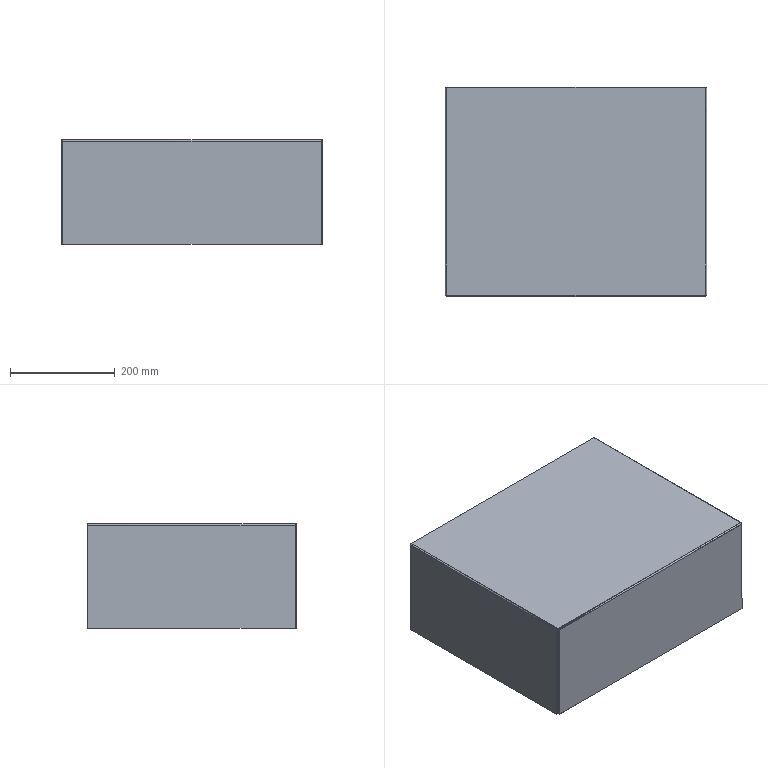Component | SolidWorks | Guard-1 | 1 solid | 30 faces | box 500 x 400 x 200 mm | volume 908561 mm3 | plane 20 | cylinder 6 | spline 4 | commonest cylinder face diameters 5.473 x3 1.473 x3
STEP:
#1=COLOUR_RGB('',0.7922,0.8196,0.9333);
#2=FILL_AREA_STYLE_COLOUR('',#1);
#3=FILL_AREA_STYLE('',(#2));
#4=SURFACE_STYLE_FILL_AREA(#3);
#5=SURFACE_SIDE_STYLE('',(#4));
#6=SURFACE_STYLE_USAGE(.BOTH.,#5);
#7=PRESENTATION_STYLE_ASSIGNMENT((#6));
#8=CARTESIAN_POINT('',(10.744,-9.76,24.528));
#9=VERTEX_POINT('',#8);
#10=CARTESIAN_POINT('',(-8.726,-9.76,24.528));
#11=VERTEX_POINT('',#10);
#12=CARTESIAN_POINT('',(-8.833,-9.76,24.528));
#13=DIRECTION('',(-1.,0.,0.));
#14=VECTOR('',#13,39.37);
#15=LINE('',#12,#14);
#16=EDGE_CURVE('',#9,#11,#15,.T.);
#17=ORIENTED_EDGE('',*,*,#16,.F.);
#18=CARTESIAN_POINT('',(10.744,-25.4,24.528));
#19=VERTEX_POINT('',#18);
#20=CARTESIAN_POINT('',(10.744,-25.401,24.528));
#21=DIRECTION('',(0.,1.,0.));
#22=VECTOR('',#21,39.37);
#23=LINE('',#20,#22);
#24=EDGE_CURVE('',#19,#9,#23,.T.);
#25=ORIENTED_EDGE('',*,*,#24,.F.);
#26=CARTESIAN_POINT('',(-8.726,-25.4,24.528));
#27=VERTEX_POINT('',#26);
#28=CARTESIAN_POINT('',(-8.727,-25.4,24.528));
#29=DIRECTION('',(1.,0.,0.));
#30=VECTOR('',#29,39.37);
#31=LINE('',#28,#30);
#32=EDGE_CURVE('',#27,#19,#31,.T.);
#33=ORIENTED_EDGE('',*,*,#32,.F.);
#34=CARTESIAN_POINT('',(-8.726,-9.76,24.528));
#35=DIRECTION('',(0.,-1.,0.));
#36=VECTOR('',#35,39.37);
#37=LINE('',#34,#36);
#38=EDGE_CURVE('',#11,#27,#37,.T.);
#39=ORIENTED_EDGE('',*,*,#38,.F.);
#40=EDGE_LOOP('',(#17,#25,#33,#39));
#41=FACE_OUTER_BOUND('',#40,.T.);
#42=CARTESIAN_POINT('',(1.009,-17.634,24.528));
#43=DIRECTION('',(0.,0.,-1.));
#44=DIRECTION('',(-1.,0.,0.));
#45=AXIS2_PLACEMENT_3D('',#42,#43,#44);
#46=PLANE('',#45);
#47=ADVANCED_FACE('',(#41),#46,.T.);
#48=CARTESIAN_POINT('',(10.744,-25.4,24.606));
#49=VERTEX_POINT('',#48);
#50=CARTESIAN_POINT('',(10.744,-9.76,24.606));
#51=VERTEX_POINT('',#50);
#52=CARTESIAN_POINT('',(10.744,-25.401,24.606));
#53=DIRECTION('',(0.,1.,0.));
#54=VECTOR('',#53,39.37);
#55=LINE('',#52,#54);
#56=EDGE_CURVE('',#49,#51,#55,.T.);
#57=ORIENTED_EDGE('',*,*,#56,.T.);
#58=CARTESIAN_POINT('',(-8.726,-9.76,24.606));
#59=VERTEX_POINT('',#58);
#60=CARTESIAN_POINT('',(-8.833,-9.76,24.606));
#61=DIRECTION('',(-1.,0.,0.));
#62=VECTOR('',#61,39.37);
#63=LINE('',#60,#62);
#64=EDGE_CURVE('',#51,#59,#63,.T.);
#65=ORIENTED_EDGE('',*,*,#64,.T.);
#66=CARTESIAN_POINT('',(-8.726,-25.4,24.606));
#67=VERTEX_POINT('',#66);
#68=CARTESIAN_POINT('',(-8.726,-9.76,24.606));
#69=DIRECTION('',(0.,-1.,0.));
#70=VECTOR('',#69,39.37);
#71=LINE('',#68,#70);
#72=EDGE_CURVE('',#59,#67,#71,.T.);
#73=ORIENTED_EDGE('',*,*,#72,.T.);
#74=CARTESIAN_POINT('',(-8.727,-25.4,24.606));
#75=DIRECTION('',(1.,0.,0.));
#76=VECTOR('',#75,39.37);
#77=LINE('',#74,#76);
#78=EDGE_CURVE('',#67,#49,#77,.T.);
#79=ORIENTED_EDGE('',*,*,#78,.T.);
#80=EDGE_LOOP('',(#57,#65,#73,#79));
#81=FACE_OUTER_BOUND('',#80,.T.);
#82=CARTESIAN_POINT('',(1.009,-17.634,24.606));
#83=DIRECTION('',(0.,0.,-1.));
#84=DIRECTION('',(-1.,0.,0.));
#85=AXIS2_PLACEMENT_3D('',#82,#83,#84);
#86=PLANE('',#85);
#87=ADVANCED_FACE('',(#81),#86,.F.);
#88=CARTESIAN_POINT('',(10.744,-9.76,24.528));
#89=DIRECTION('',(0.,0.,1.));
#90=VECTOR('',#89,39.37);
#91=LINE('',#88,#90);
#92=EDGE_CURVE('',#9,#51,#91,.T.);
#93=ORIENTED_EDGE('',*,*,#92,.F.);
#94=ORIENTED_EDGE('',*,*,#16,.T.);
#95=CARTESIAN_POINT('',(-8.726,-9.76,24.528));
#96=DIRECTION('',(0.,0.,1.));
#97=VECTOR('',#96,39.37);
#98=LINE('',#95,#97);
#99=EDGE_CURVE('',#11,#59,#98,.T.);
#100=ORIENTED_EDGE('',*,*,#99,.T.);
#101=ORIENTED_EDGE('',*,*,#64,.F.);
#102=EDGE_LOOP('',(#93,#94,#100,#101));
#103=FACE_OUTER_BOUND('',#102,.T.);
#104=CARTESIAN_POINT('',(-8.833,-9.76,24.528));
#105=DIRECTION('',(0.,1.,0.));
#106=DIRECTION('',(0.,0.,1.));
#107=AXIS2_PLACEMENT_3D('',#104,#105,#106);
#108=PLANE('',#107);
#109=ADVANCED_FACE('',(#103),#108,.T.);
#110=CARTESIAN_POINT('',(-8.833,-25.401,24.499));
#111=VERTEX_POINT('',#110);
#112=CARTESIAN_POINT('',(-8.755,-25.401,24.499));
#113=VERTEX_POINT('',#112);
#114=CARTESIAN_POINT('',(-8.755,-25.401,24.499));
#115=DIRECTION('',(1.,0.,-0.));
#116=VECTOR('',#115,39.37);
#117=LINE('',#114,#116);
#118=EDGE_CURVE('',#111,#113,#117,.T.);
#119=ORIENTED_EDGE('',*,*,#118,.T.);
#120=CARTESIAN_POINT('',(-8.726,-25.4,24.528));
#121=CARTESIAN_POINT('',(-8.733,-25.4,24.528));
#122=CARTESIAN_POINT('',(-8.741,-25.401,24.524));
#123=CARTESIAN_POINT('',(-8.752,-25.401,24.514));
#124=CARTESIAN_POINT('',(-8.755,-25.401,24.506));
#125=CARTESIAN_POINT('',(-8.755,-25.401,24.499));
#126=B_SPLINE_CURVE_WITH_KNOTS('',3,(#120,#121,#122,#123,#124,#125),.UNSPECIFIED.,.F.,.F.,(4,2,4),(0.,0.5,1.),.UNSPECIFIED.);
#127=EDGE_CURVE('',#27,#113,#126,.T.);
#128=ORIENTED_EDGE('',*,*,#127,.F.);
#129=CARTESIAN_POINT('',(-8.726,-25.4,24.528));
#130=DIRECTION('',(0.,0.,1.));
#131=VECTOR('',#130,39.37);
#132=LINE('',#129,#131);
#133=EDGE_CURVE('',#27,#67,#132,.T.);
#134=ORIENTED_EDGE('',*,*,#133,.T.);
#135=CARTESIAN_POINT('',(-8.726,-25.4,24.606));
#136=CARTESIAN_POINT('',(-8.74,-25.4,24.606));
#137=CARTESIAN_POINT('',(-8.754,-25.4,24.603));
#138=CARTESIAN_POINT('',(-8.78,-25.401,24.593));
#139=CARTESIAN_POINT('',(-8.792,-25.401,24.585));
#140=CARTESIAN_POINT('',(-8.812,-25.401,24.565));
#141=CARTESIAN_POINT('',(-8.82,-25.401,24.553));
#142=CARTESIAN_POINT('',(-8.831,-25.401,24.527));
#143=CARTESIAN_POINT('',(-8.833,-25.401,24.513));
#144=CARTESIAN_POINT('',(-8.833,-25.401,24.499));
#145=B_SPLINE_CURVE_WITH_KNOTS('',3,(#135,#136,#137,#138,#139,#140,#141,#142,#143,#144),.UNSPECIFIED.,.F.,.F.,(4,2,2,2,4),(0.,0.25,0.5,0.75,1.),.UNSPECIFIED.);
#146=EDGE_CURVE('',#67,#111,#145,.T.);
#147=ORIENTED_EDGE('',*,*,#146,.T.);
#148=EDGE_LOOP('',(#119,#128,#134,#147));
#149=FACE_OUTER_BOUND('',#148,.T.);
#150=CARTESIAN_POINT('',(-8.726,-25.4,24.607));
#151=CARTESIAN_POINT('',(-8.74,-25.4,24.607));
#152=CARTESIAN_POINT('',(-8.754,-25.4,24.604));
#153=CARTESIAN_POINT('',(-8.78,-25.401,24.593));
#154=CARTESIAN_POINT('',(-8.792,-25.401,24.585));
#155=CARTESIAN_POINT('',(-8.813,-25.401,24.565));
#156=CARTESIAN_POINT('',(-8.821,-25.401,24.553));
#157=CARTESIAN_POINT('',(-8.831,-25.401,24.527));
#158=CARTESIAN_POINT('',(-8.834,-25.401,24.513));
#159=CARTESIAN_POINT('',(-8.834,-25.401,24.499));
#160=CARTESIAN_POINT('',(-8.726,-25.4,24.606));
#161=CARTESIAN_POINT('',(-8.74,-25.4,24.606));
#162=CARTESIAN_POINT('',(-8.754,-25.4,24.603));
#163=CARTESIAN_POINT('',(-8.78,-25.401,24.593));
#164=CARTESIAN_POINT('',(-8.792,-25.401,24.585));
#165=CARTESIAN_POINT('',(-8.812,-25.401,24.565));
#166=CARTESIAN_POINT('',(-8.82,-25.401,24.553));
#167=CARTESIAN_POINT('',(-8.831,-25.401,24.527));
#168=CARTESIAN_POINT('',(-8.833,-25.401,24.513));
#169=CARTESIAN_POINT('',(-8.833,-25.401,24.499));
#170=CARTESIAN_POINT('',(-8.726,-25.4,24.528));
#171=CARTESIAN_POINT('',(-8.73,-25.4,24.528));
#172=CARTESIAN_POINT('',(-8.733,-25.4,24.527));
#173=CARTESIAN_POINT('',(-8.74,-25.401,24.524));
#174=CARTESIAN_POINT('',(-8.744,-25.401,24.522));
#175=CARTESIAN_POINT('',(-8.749,-25.401,24.516));
#176=CARTESIAN_POINT('',(-8.751,-25.401,24.513));
#177=CARTESIAN_POINT('',(-8.754,-25.401,24.506));
#178=CARTESIAN_POINT('',(-8.755,-25.401,24.502));
#179=CARTESIAN_POINT('',(-8.755,-25.401,24.499));
#180=CARTESIAN_POINT('',(-8.726,-25.4,24.527));
#181=CARTESIAN_POINT('',(-8.729,-25.4,24.527));
#182=CARTESIAN_POINT('',(-8.733,-25.4,24.526));
#183=CARTESIAN_POINT('',(-8.74,-25.401,24.523));
#184=CARTESIAN_POINT('',(-8.743,-25.401,24.521));
#185=CARTESIAN_POINT('',(-8.748,-25.401,24.516));
#186=CARTESIAN_POINT('',(-8.75,-25.401,24.513));
#187=CARTESIAN_POINT('',(-8.753,-25.401,24.506));
#188=CARTESIAN_POINT('',(-8.754,-25.401,24.502));
#189=CARTESIAN_POINT('',(-8.754,-25.401,24.499));
#190=B_SPLINE_SURFACE_WITH_KNOTS('',1,3,((#150,#151,#152,#153,#154,#155,#156,#157,#158,#159),(#160,#161,#162,#163,#164,#165,#166,#167,#168,#169),(#170,#171,#172,#173,#174,#175,#176,#177,#178,#179),(#180,#181,#182,#183,#184,#185,#186,#187,#188,#189)),.UNSPECIFIED.,.F.,.F.,.F.,(2,1,1,2),(4,2,2,2,4),(-0.01,0.,1.,1.01),(0.,0.25,0.5,0.75,1.),.UNSPECIFIED.);
#191=ADVANCED_FACE('',(#149),#190,.F.);
#192=CARTESIAN_POINT('',(-8.755,-9.76,24.499));
#193=VERTEX_POINT('',#192);
#194=CARTESIAN_POINT('',(-8.726,-9.76,24.499));
#195=DIRECTION('',(0.,1.,0.));
#196=DIRECTION('',(0.,0.,1.));
#197=AXIS2_PLACEMENT_3D('',#194,#195,#196);
#198=CIRCLE('',#197,0.029);
#199=EDGE_CURVE('',#193,#11,#198,.T.);
#200=ORIENTED_EDGE('',*,*,#199,.F.);
#201=CARTESIAN_POINT('',(-8.833,-9.76,24.499));
#202=VERTEX_POINT('',#201);
#203=CARTESIAN_POINT('',(-8.755,-9.76,24.499));
#204=DIRECTION('',(-1.,0.,0.));
#205=VECTOR('',#204,39.37);
#206=LINE('',#203,#205);
#207=EDGE_CURVE('',#193,#202,#206,.T.);
#208=ORIENTED_EDGE('',*,*,#207,.T.);
#209=CARTESIAN_POINT('',(-8.726,-9.76,24.499));
#210=DIRECTION('',(0.,1.,0.));
#211=DIRECTION('',(0.,0.,1.));
#212=AXIS2_PLACEMENT_3D('',#209,#210,#211);
#213=CIRCLE('',#212,0.1077);
#214=EDGE_CURVE('',#202,#59,#213,.T.);
#215=ORIENTED_EDGE('',*,*,#214,.T.);
#216=ORIENTED_EDGE('',*,*,#99,.F.);
#217=EDGE_LOOP('',(#200,#208,#215,#216));
#218=FACE_OUTER_BOUND('',#217,.T.);
#219=CARTESIAN_POINT('',(-8.726,-9.76,24.499));
#220=DIRECTION('',(0.,-1.,0.));
#221=DIRECTION('',(0.,0.,-1.));
#222=AXIS2_PLACEMENT_3D('',#219,#220,#221);
#223=PLANE('',#222);
#224=ADVANCED_FACE('',(#218),#223,.F.);
#225=ORIENTED_EDGE('',*,*,#72,.F.);
#226=ORIENTED_EDGE('',*,*,#214,.F.);
#227=CARTESIAN_POINT('',(-8.833,-17.634,24.499));
#228=DIRECTION('',(0.,1.,0.));
#229=VECTOR('',#228,39.37);
#230=LINE('',#227,#229);
#231=EDGE_CURVE('',#111,#202,#230,.T.);
#232=ORIENTED_EDGE('',*,*,#231,.F.);
#233=ORIENTED_EDGE('',*,*,#146,.F.);
#234=EDGE_LOOP('',(#225,#226,#232,#233));
#235=FACE_OUTER_BOUND('',#234,.T.);
#236=CARTESIAN_POINT('',(-8.726,-9.76,24.499));
#237=DIRECTION('',(0.,1.,0.));
#238=DIRECTION('',(-1.,0.,0.));
#239=AXIS2_PLACEMENT_3D('',#236,#237,#238);
#240=CYLINDRICAL_SURFACE('',#239,0.1077);
#241=ADVANCED_FACE('',(#235),#240,.T.);
#242=ORIENTED_EDGE('',*,*,#38,.T.);
#243=ORIENTED_EDGE('',*,*,#127,.T.);
#244=CARTESIAN_POINT('',(-8.755,-25.508,24.499));
#245=DIRECTION('',(0.,1.,0.));
#246=VECTOR('',#245,39.37);
#247=LINE('',#244,#246);
#248=EDGE_CURVE('',#113,#193,#247,.T.);
#249=ORIENTED_EDGE('',*,*,#248,.T.);
#250=ORIENTED_EDGE('',*,*,#199,.T.);
#251=EDGE_LOOP('',(#242,#243,#249,#250));
#252=FACE_OUTER_BOUND('',#251,.T.);
#253=CARTESIAN_POINT('',(-8.726,-9.76,24.499));
#254=DIRECTION('',(0.,1.,0.));
#255=DIRECTION('',(-1.,0.,0.));
#256=AXIS2_PLACEMENT_3D('',#253,#254,#255);
#257=CYLINDRICAL_SURFACE('',#256,0.029);
#258=ADVANCED_FACE('',(#252),#257,.F.);
#259=CARTESIAN_POINT('',(-8.755,-25.401,16.732));
#260=VERTEX_POINT('',#259);
#261=CARTESIAN_POINT('',(-8.833,-25.401,16.732));
#262=VERTEX_POINT('',#261);
#263=CARTESIAN_POINT('',(-8.833,-25.401,16.732));
#264=DIRECTION('',(-1.,-0.,0.));
#265=VECTOR('',#264,39.37);
#266=LINE('',#263,#265);
#267=EDGE_CURVE('',#260,#262,#266,.T.);
#268=ORIENTED_EDGE('',*,*,#267,.F.);
#269=CARTESIAN_POINT('',(-8.755,-25.401,24.606));
#270=DIRECTION('',(-0.,0.,-1.));
#271=VECTOR('',#270,39.37);
#272=LINE('',#269,#271);
#273=EDGE_CURVE('',#113,#260,#272,.T.);
#274=ORIENTED_EDGE('',*,*,#273,.F.);
#275=ORIENTED_EDGE('',*,*,#118,.F.);
#276=CARTESIAN_POINT('',(-8.833,-25.401,24.606));
#277=DIRECTION('',(0.,-0.,1.));
#278=VECTOR('',#277,39.37);
#279=LINE('',#276,#278);
#280=EDGE_CURVE('',#262,#111,#279,.T.);
#281=ORIENTED_EDGE('',*,*,#280,.F.);
#282=EDGE_LOOP('',(#268,#274,#275,#281));
#283=FACE_OUTER_BOUND('',#282,.T.);
#284=CARTESIAN_POINT('',(-8.755,-25.401,24.528));
#285=DIRECTION('',(-0.,-1.,-0.));
#286=DIRECTION('',(0.,0.,-1.));
#287=AXIS2_PLACEMENT_3D('',#284,#285,#286);
#288=PLANE('',#287);
#289=ADVANCED_FACE('',(#283),#288,.T.);
#290=CARTESIAN_POINT('',(-8.833,-9.76,16.732));
#291=VERTEX_POINT('',#290);
#292=CARTESIAN_POINT('',(-8.833,-9.76,16.732));
#293=DIRECTION('',(0.,1.,0.));
#294=VECTOR('',#293,39.37);
#295=LINE('',#292,#294);
#296=EDGE_CURVE('',#262,#291,#295,.T.);
#297=ORIENTED_EDGE('',*,*,#296,.F.);
#298=ORIENTED_EDGE('',*,*,#280,.T.);
#299=ORIENTED_EDGE('',*,*,#231,.T.);
#300=CARTESIAN_POINT('',(-8.833,-9.76,24.528));
#301=DIRECTION('',(0.,0.,1.));
#302=VECTOR('',#301,39.37);
#303=LINE('',#300,#302);
#304=EDGE_CURVE('',#291,#202,#303,.T.);
#305=ORIENTED_EDGE('',*,*,#304,.F.);
#306=EDGE_LOOP('',(#297,#298,#299,#305));
#307=FACE_OUTER_BOUND('',#306,.T.);
#308=CARTESIAN_POINT('',(-8.833,-17.634,24.606));
#309=DIRECTION('',(-1.,0.,0.));
#310=DIRECTION('',(0.,0.,1.));
#311=AXIS2_PLACEMENT_3D('',#308,#309,#310);
#312=PLANE('',#311);
#313=ADVANCED_FACE('',(#307),#312,.T.);
#314=ORIENTED_EDGE('',*,*,#273,.T.);
#315=CARTESIAN_POINT('',(-8.755,-9.76,16.732));
#316=VERTEX_POINT('',#315);
#317=CARTESIAN_POINT('',(-8.755,-17.634,16.732));
#318=DIRECTION('',(0.,1.,0.));
#319=VECTOR('',#318,39.37);
#320=LINE('',#317,#319);
#321=EDGE_CURVE('',#260,#316,#320,.T.);
#322=ORIENTED_EDGE('',*,*,#321,.T.);
#323=CARTESIAN_POINT('',(-8.755,-9.76,24.606));
#324=DIRECTION('',(0.,0.,1.));
#325=VECTOR('',#324,39.37);
#326=LINE('',#323,#325);
#327=EDGE_CURVE('',#316,#193,#326,.T.);
#328=ORIENTED_EDGE('',*,*,#327,.T.);
#329=ORIENTED_EDGE('',*,*,#248,.F.);
#330=EDGE_LOOP('',(#314,#322,#328,#329));
#331=FACE_OUTER_BOUND('',#330,.T.);
#332=CARTESIAN_POINT('',(-8.755,-17.634,24.606));
#333=DIRECTION('',(-1.,0.,0.));
#334=DIRECTION('',(0.,0.,1.));
#335=AXIS2_PLACEMENT_3D('',#332,#333,#334);
#336=PLANE('',#335);
#337=ADVANCED_FACE('',(#331),#336,.F.);
#338=ORIENTED_EDGE('',*,*,#321,.F.);
#339=ORIENTED_EDGE('',*,*,#267,.T.);
#340=ORIENTED_EDGE('',*,*,#296,.T.);
#341=CARTESIAN_POINT('',(-8.833,-9.76,16.732));
#342=DIRECTION('',(1.,0.,-0.));
#343=VECTOR('',#342,39.37);
#344=LINE('',#341,#343);
#345=EDGE_CURVE('',#291,#316,#344,.T.);
#346=ORIENTED_EDGE('',*,*,#345,.T.);
#347=EDGE_LOOP('',(#338,#339,#340,#346));
#348=FACE_OUTER_BOUND('',#347,.T.);
#349=CARTESIAN_POINT('',(-8.833,-9.76,16.732));
#350=DIRECTION('',(-0.,0.,-1.));
#351=DIRECTION('',(-1.,0.,0.));
#352=AXIS2_PLACEMENT_3D('',#349,#350,#351);
#353=PLANE('',#352);
#354=ADVANCED_FACE('',(#348),#353,.T.);
#355=ORIENTED_EDGE('',*,*,#304,.T.);
#356=ORIENTED_EDGE('',*,*,#207,.F.);
#357=ORIENTED_EDGE('',*,*,#327,.F.);
#358=ORIENTED_EDGE('',*,*,#345,.F.);
#359=EDGE_LOOP('',(#355,#356,#357,#358));
#360=FACE_OUTER_BOUND('',#359,.T.);
#361=CARTESIAN_POINT('',(-8.833,-9.76,24.528));
#362=DIRECTION('',(0.,1.,0.));
#363=DIRECTION('',(0.,0.,1.));
#364=AXIS2_PLACEMENT_3D('',#361,#362,#363);
#365=PLANE('',#364);
#366=ADVANCED_FACE('',(#360),#365,.T.);
#367=CARTESIAN_POINT('',(10.745,-25.508,24.499));
#368=VERTEX_POINT('',#367);
#369=CARTESIAN_POINT('',(10.745,-25.429,24.499));
#370=VERTEX_POINT('',#369);
#371=CARTESIAN_POINT('',(10.745,-25.429,24.499));
#372=DIRECTION('',(0.,1.,-0.));
#373=VECTOR('',#372,39.37);
#374=LINE('',#371,#373);
#375=EDGE_CURVE('',#368,#370,#374,.T.);
#376=ORIENTED_EDGE('',*,*,#375,.T.);
#377=CARTESIAN_POINT('',(10.744,-25.4,24.528));
#378=CARTESIAN_POINT('',(10.744,-25.408,24.528));
#379=CARTESIAN_POINT('',(10.744,-25.415,24.524));
#380=CARTESIAN_POINT('',(10.745,-25.426,24.514));
#381=CARTESIAN_POINT('',(10.745,-25.429,24.506));
#382=CARTESIAN_POINT('',(10.745,-25.429,24.499));
#383=B_SPLINE_CURVE_WITH_KNOTS('',3,(#377,#378,#379,#380,#381,#382),.UNSPECIFIED.,.F.,.F.,(4,2,4),(0.,0.5,1.),.UNSPECIFIED.);
#384=EDGE_CURVE('',#19,#370,#383,.T.);
#385=ORIENTED_EDGE('',*,*,#384,.F.);
#386=CARTESIAN_POINT('',(10.744,-25.4,24.528));
#387=DIRECTION('',(0.,0.,1.));
#388=VECTOR('',#387,39.37);
#389=LINE('',#386,#388);
#390=EDGE_CURVE('',#19,#49,#389,.T.);
#391=ORIENTED_EDGE('',*,*,#390,.T.);
#392=CARTESIAN_POINT('',(10.744,-25.4,24.606));
#393=CARTESIAN_POINT('',(10.744,-25.414,24.606));
#394=CARTESIAN_POINT('',(10.744,-25.428,24.603));
#395=CARTESIAN_POINT('',(10.744,-25.454,24.593));
#396=CARTESIAN_POINT('',(10.744,-25.466,24.585));
#397=CARTESIAN_POINT('',(10.744,-25.486,24.565));
#398=CARTESIAN_POINT('',(10.745,-25.494,24.553));
#399=CARTESIAN_POINT('',(10.745,-25.505,24.527));
#400=CARTESIAN_POINT('',(10.745,-25.508,24.513));
#401=CARTESIAN_POINT('',(10.745,-25.508,24.499));
#402=B_SPLINE_CURVE_WITH_KNOTS('',3,(#392,#393,#394,#395,#396,#397,#398,#399,#400,#401),.UNSPECIFIED.,.F.,.F.,(4,2,2,2,4),(0.,0.25,0.5,0.75,1.),.UNSPECIFIED.);
#403=EDGE_CURVE('',#49,#368,#402,.T.);
#404=ORIENTED_EDGE('',*,*,#403,.T.);
#405=EDGE_LOOP('',(#376,#385,#391,#404));
#406=FACE_OUTER_BOUND('',#405,.T.);
#407=CARTESIAN_POINT('',(10.744,-25.4,24.607));
#408=CARTESIAN_POINT('',(10.744,-25.414,24.607));
#409=CARTESIAN_POINT('',(10.744,-25.429,24.604));
#410=CARTESIAN_POINT('',(10.744,-25.455,24.593));
#411=CARTESIAN_POINT('',(10.744,-25.467,24.585));
#412=CARTESIAN_POINT('',(10.744,-25.487,24.565));
#413=CARTESIAN_POINT('',(10.745,-25.495,24.553));
#414=CARTESIAN_POINT('',(10.745,-25.506,24.527));
#415=CARTESIAN_POINT('',(10.745,-25.509,24.513));
#416=CARTESIAN_POINT('',(10.745,-25.509,24.499));
#417=CARTESIAN_POINT('',(10.744,-25.4,24.606));
#418=CARTESIAN_POINT('',(10.744,-25.414,24.606));
#419=CARTESIAN_POINT('',(10.744,-25.428,24.603));
#420=CARTESIAN_POINT('',(10.744,-25.454,24.593));
#421=CARTESIAN_POINT('',(10.744,-25.466,24.585));
#422=CARTESIAN_POINT('',(10.744,-25.486,24.565));
#423=CARTESIAN_POINT('',(10.745,-25.494,24.553));
#424=CARTESIAN_POINT('',(10.745,-25.505,24.527));
#425=CARTESIAN_POINT('',(10.745,-25.508,24.513));
#426=CARTESIAN_POINT('',(10.745,-25.508,24.499));
#427=CARTESIAN_POINT('',(10.744,-25.4,24.528));
#428=CARTESIAN_POINT('',(10.744,-25.404,24.528));
#429=CARTESIAN_POINT('',(10.744,-25.408,24.527));
#430=CARTESIAN_POINT('',(10.744,-25.415,24.524));
#431=CARTESIAN_POINT('',(10.744,-25.418,24.522));
#432=CARTESIAN_POINT('',(10.744,-25.423,24.516));
#433=CARTESIAN_POINT('',(10.745,-25.425,24.513));
#434=CARTESIAN_POINT('',(10.745,-25.428,24.506));
#435=CARTESIAN_POINT('',(10.745,-25.429,24.502));
#436=CARTESIAN_POINT('',(10.745,-25.429,24.499));
#437=CARTESIAN_POINT('',(10.744,-25.4,24.527));
#438=CARTESIAN_POINT('',(10.744,-25.404,24.527));
#439=CARTESIAN_POINT('',(10.744,-25.408,24.526));
#440=CARTESIAN_POINT('',(10.744,-25.414,24.523));
#441=CARTESIAN_POINT('',(10.744,-25.417,24.521));
#442=CARTESIAN_POINT('',(10.744,-25.423,24.516));
#443=CARTESIAN_POINT('',(10.745,-25.425,24.513));
#444=CARTESIAN_POINT('',(10.745,-25.428,24.506));
#445=CARTESIAN_POINT('',(10.745,-25.428,24.502));
#446=CARTESIAN_POINT('',(10.745,-25.428,24.499));
#447=B_SPLINE_SURFACE_WITH_KNOTS('',1,3,((#407,#408,#409,#410,#411,#412,#413,#414,#415,#416),(#417,#418,#419,#420,#421,#422,#423,#424,#425,#426),(#427,#428,#429,#430,#431,#432,#433,#434,#435,#436),(#437,#438,#439,#440,#441,#442,#443,#444,#445,#446)),.UNSPECIFIED.,.F.,.F.,.F.,(2,1,1,2),(4,2,2,2,4),(-0.01,0.,1.,1.01),(0.,0.25,0.5,0.75,1.),.UNSPECIFIED.);
#448=ADVANCED_FACE('',(#406),#447,.F.);
#449=CARTESIAN_POINT('',(-8.727,-25.429,24.499));
#450=VERTEX_POINT('',#449);
#451=CARTESIAN_POINT('',(-8.727,-25.429,24.499));
#452=CARTESIAN_POINT('',(-8.727,-25.429,24.506));
#453=CARTESIAN_POINT('',(-8.727,-25.426,24.514));
#454=CARTESIAN_POINT('',(-8.726,-25.415,24.524));
#455=CARTESIAN_POINT('',(-8.726,-25.408,24.528));
#456=CARTESIAN_POINT('',(-8.726,-25.4,24.528));
#457=B_SPLINE_CURVE_WITH_KNOTS('',3,(#451,#452,#453,#454,#455,#456),.UNSPECIFIED.,.F.,.F.,(4,2,4),(0.,0.5,1.),.UNSPECIFIED.);
#458=EDGE_CURVE('',#450,#27,#457,.T.);
#459=ORIENTED_EDGE('',*,*,#458,.F.);
#460=CARTESIAN_POINT('',(-8.727,-25.508,24.499));
#461=VERTEX_POINT('',#460);
#462=CARTESIAN_POINT('',(-8.727,-25.429,24.499));
#463=DIRECTION('',(0.,1.,-0.));
#464=VECTOR('',#463,39.37);
#465=LINE('',#462,#464);
#466=EDGE_CURVE('',#461,#450,#465,.T.);
#467=ORIENTED_EDGE('',*,*,#466,.F.);
#468=CARTESIAN_POINT('',(-8.727,-25.508,24.499));
#469=CARTESIAN_POINT('',(-8.727,-25.508,24.513));
#470=CARTESIAN_POINT('',(-8.727,-25.505,24.527));
#471=CARTESIAN_POINT('',(-8.727,-25.494,24.553));
#472=CARTESIAN_POINT('',(-8.726,-25.486,24.565));
#473=CARTESIAN_POINT('',(-8.726,-25.466,24.585));
#474=CARTESIAN_POINT('',(-8.726,-25.454,24.593));
#475=CARTESIAN_POINT('',(-8.726,-25.428,24.603));
#476=CARTESIAN_POINT('',(-8.726,-25.414,24.606));
#477=CARTESIAN_POINT('',(-8.726,-25.4,24.606));
#478=B_SPLINE_CURVE_WITH_KNOTS('',3,(#468,#469,#470,#471,#472,#473,#474,#475,#476,#477),.UNSPECIFIED.,.F.,.F.,(4,2,2,2,4),(0.,0.25,0.5,0.75,1.),.UNSPECIFIED.);
#479=EDGE_CURVE('',#461,#67,#478,.T.);
#480=ORIENTED_EDGE('',*,*,#479,.T.);
#481=ORIENTED_EDGE('',*,*,#133,.F.);
#482=EDGE_LOOP('',(#459,#467,#480,#481));
#483=FACE_OUTER_BOUND('',#482,.T.);
#484=CARTESIAN_POINT('',(-8.727,-25.509,24.499));
#485=CARTESIAN_POINT('',(-8.727,-25.509,24.513));
#486=CARTESIAN_POINT('',(-8.727,-25.506,24.527));
#487=CARTESIAN_POINT('',(-8.727,-25.495,24.553));
#488=CARTESIAN_POINT('',(-8.726,-25.487,24.565));
#489=CARTESIAN_POINT('',(-8.726,-25.467,24.585));
#490=CARTESIAN_POINT('',(-8.726,-25.455,24.593));
#491=CARTESIAN_POINT('',(-8.726,-25.429,24.604));
#492=CARTESIAN_POINT('',(-8.726,-25.414,24.607));
#493=CARTESIAN_POINT('',(-8.726,-25.4,24.607));
#494=CARTESIAN_POINT('',(-8.727,-25.508,24.499));
#495=CARTESIAN_POINT('',(-8.727,-25.508,24.513));
#496=CARTESIAN_POINT('',(-8.727,-25.505,24.527));
#497=CARTESIAN_POINT('',(-8.727,-25.494,24.553));
#498=CARTESIAN_POINT('',(-8.726,-25.486,24.565));
#499=CARTESIAN_POINT('',(-8.726,-25.466,24.585));
#500=CARTESIAN_POINT('',(-8.726,-25.454,24.593));
#501=CARTESIAN_POINT('',(-8.726,-25.428,24.603));
#502=CARTESIAN_POINT('',(-8.726,-25.414,24.606));
#503=CARTESIAN_POINT('',(-8.726,-25.4,24.606));
#504=CARTESIAN_POINT('',(-8.727,-25.429,24.499));
#505=CARTESIAN_POINT('',(-8.727,-25.429,24.502));
#506=CARTESIAN_POINT('',(-8.727,-25.428,24.506));
#507=CARTESIAN_POINT('',(-8.727,-25.425,24.513));
#508=CARTESIAN_POINT('',(-8.726,-25.423,24.516));
#509=CARTESIAN_POINT('',(-8.726,-25.418,24.522));
#510=CARTESIAN_POINT('',(-8.726,-25.415,24.524));
#511=CARTESIAN_POINT('',(-8.726,-25.408,24.527));
#512=CARTESIAN_POINT('',(-8.726,-25.404,24.528));
#513=CARTESIAN_POINT('',(-8.726,-25.4,24.528));
#514=CARTESIAN_POINT('',(-8.727,-25.428,24.499));
#515=CARTESIAN_POINT('',(-8.727,-25.428,24.502));
#516=CARTESIAN_POINT('',(-8.727,-25.428,24.506));
#517=CARTESIAN_POINT('',(-8.727,-25.425,24.513));
#518=CARTESIAN_POINT('',(-8.726,-25.423,24.516));
#519=CARTESIAN_POINT('',(-8.726,-25.417,24.521));
#520=CARTESIAN_POINT('',(-8.726,-25.414,24.523));
#521=CARTESIAN_POINT('',(-8.726,-25.408,24.526));
#522=CARTESIAN_POINT('',(-8.726,-25.404,24.527));
#523=CARTESIAN_POINT('',(-8.726,-25.4,24.527));
#524=B_SPLINE_SURFACE_WITH_KNOTS('',1,3,((#484,#485,#486,#487,#488,#489,#490,#491,#492,#493),(#494,#495,#496,#497,#498,#499,#500,#501,#502,#503),(#504,#505,#506,#507,#508,#509,#510,#511,#512,#513),(#514,#515,#516,#517,#518,#519,#520,#521,#522,#523)),.UNSPECIFIED.,.F.,.F.,.F.,(2,1,1,2),(4,2,2,2,4),(-0.01,0.,1.,1.01),(0.,0.25,0.5,0.75,1.),.UNSPECIFIED.);
#525=ADVANCED_FACE('',(#483),#524,.F.);
#526=ORIENTED_EDGE('',*,*,#78,.F.);
#527=ORIENTED_EDGE('',*,*,#479,.F.);
#528=CARTESIAN_POINT('',(10.852,-25.508,24.499));
#529=DIRECTION('',(1.,0.,0.));
#530=VECTOR('',#529,39.37);
#531=LINE('',#528,#530);
#532=EDGE_CURVE('',#461,#368,#531,.T.);
#533=ORIENTED_EDGE('',*,*,#532,.T.);
#534=ORIENTED_EDGE('',*,*,#403,.F.);
#535=EDGE_LOOP('',(#526,#527,#533,#534));
#536=FACE_OUTER_BOUND('',#535,.T.);
#537=CARTESIAN_POINT('',(-8.727,-25.4,24.499));
#538=DIRECTION('',(-1.,0.,0.));
#539=DIRECTION('',(0.,-1.,0.));
#540=AXIS2_PLACEMENT_3D('',#537,#538,#539);
#541=CYLINDRICAL_SURFACE('',#540,0.1077);
#542=ADVANCED_FACE('',(#536),#541,.T.);
#543=ORIENTED_EDGE('',*,*,#32,.T.);
#544=ORIENTED_EDGE('',*,*,#384,.T.);
#545=CARTESIAN_POINT('',(10.852,-25.429,24.499));
#546=DIRECTION('',(-1.,0.,0.));
#547=VECTOR('',#546,39.37);
#548=LINE('',#545,#547);
#549=EDGE_CURVE('',#370,#450,#548,.T.);
#550=ORIENTED_EDGE('',*,*,#549,.T.);
#551=ORIENTED_EDGE('',*,*,#458,.T.);
#552=EDGE_LOOP('',(#543,#544,#550,#551));
#553=FACE_OUTER_BOUND('',#552,.T.);
#554=CARTESIAN_POINT('',(-8.727,-25.4,24.499));
#555=DIRECTION('',(-1.,0.,0.));
#556=DIRECTION('',(0.,-1.,0.));
#557=AXIS2_PLACEMENT_3D('',#554,#555,#556);
#558=CYLINDRICAL_SURFACE('',#557,0.029);
#559=ADVANCED_FACE('',(#553),#558,.F.);
#560=CARTESIAN_POINT('',(10.745,-25.429,16.732));
#561=VERTEX_POINT('',#560);
#562=CARTESIAN_POINT('',(10.745,-25.508,16.732));
#563=VERTEX_POINT('',#562);
#564=CARTESIAN_POINT('',(10.745,-25.508,16.732));
#565=DIRECTION('',(0.,-1.,0.));
#566=VECTOR('',#565,39.37);
#567=LINE('',#564,#566);
#568=EDGE_CURVE('',#561,#563,#567,.T.);
#569=ORIENTED_EDGE('',*,*,#568,.F.);
#570=CARTESIAN_POINT('',(10.745,-25.429,24.606));
#571=DIRECTION('',(0.,-0.,-1.));
#572=VECTOR('',#571,39.37);
#573=LINE('',#570,#572);
#574=EDGE_CURVE('',#370,#561,#573,.T.);
#575=ORIENTED_EDGE('',*,*,#574,.F.);
#576=ORIENTED_EDGE('',*,*,#375,.F.);
#577=CARTESIAN_POINT('',(10.745,-25.508,24.528));
#578=DIRECTION('',(0.,-0.,-1.));
#579=VECTOR('',#578,39.37);
#580=LINE('',#577,#579);
#581=EDGE_CURVE('',#368,#563,#580,.T.);
#582=ORIENTED_EDGE('',*,*,#581,.T.);
#583=EDGE_LOOP('',(#569,#575,#576,#582));
#584=FACE_OUTER_BOUND('',#583,.T.);
#585=CARTESIAN_POINT('',(10.745,-25.429,24.528));
#586=DIRECTION('',(1.,0.,0.));
#587=DIRECTION('',(0.,0.,-1.));
#588=AXIS2_PLACEMENT_3D('',#585,#586,#587);
#589=PLANE('',#588);
#590=ADVANCED_FACE('',(#584),#589,.T.);
#591=ORIENTED_EDGE('',*,*,#532,.F.);
#592=CARTESIAN_POINT('',(-8.727,-25.508,16.732));
#593=VERTEX_POINT('',#592);
#594=CARTESIAN_POINT('',(-8.727,-25.508,24.606));
#595=DIRECTION('',(0.,-0.,-1.));
#596=VECTOR('',#595,39.37);
#597=LINE('',#594,#596);
#598=EDGE_CURVE('',#461,#593,#597,.T.);
#599=ORIENTED_EDGE('',*,*,#598,.T.);
#600=CARTESIAN_POINT('',(10.852,-25.508,16.732));
#601=DIRECTION('',(-1.,0.,0.));
#602=VECTOR('',#601,39.37);
#603=LINE('',#600,#602);
#604=EDGE_CURVE('',#563,#593,#603,.T.);
#605=ORIENTED_EDGE('',*,*,#604,.F.);
#606=ORIENTED_EDGE('',*,*,#581,.F.);
#607=EDGE_LOOP('',(#591,#599,#605,#606));
#608=FACE_OUTER_BOUND('',#607,.T.);
#609=CARTESIAN_POINT('',(1.009,-25.508,24.606));
#610=DIRECTION('',(0.,1.,-0.));
#611=DIRECTION('',(0.,0.,1.));
#612=AXIS2_PLACEMENT_3D('',#609,#610,#611);
#613=PLANE('',#612);
#614=ADVANCED_FACE('',(#608),#613,.F.);
#615=CARTESIAN_POINT('',(-8.727,-25.429,16.732));
#616=VERTEX_POINT('',#615);
#617=CARTESIAN_POINT('',(-8.727,-25.429,24.528));
#618=DIRECTION('',(0.,-0.,-1.));
#619=VECTOR('',#618,39.37);
#620=LINE('',#617,#619);
#621=EDGE_CURVE('',#450,#616,#620,.T.);
#622=ORIENTED_EDGE('',*,*,#621,.F.);
#623=ORIENTED_EDGE('',*,*,#549,.F.);
#624=ORIENTED_EDGE('',*,*,#574,.T.);
#625=CARTESIAN_POINT('',(1.009,-25.429,16.732));
#626=DIRECTION('',(-1.,0.,0.));
#627=VECTOR('',#626,39.37);
#628=LINE('',#625,#627);
#629=EDGE_CURVE('',#561,#616,#628,.T.);
#630=ORIENTED_EDGE('',*,*,#629,.T.);
#631=EDGE_LOOP('',(#622,#623,#624,#630));
#632=FACE_OUTER_BOUND('',#631,.T.);
#633=CARTESIAN_POINT('',(1.009,-25.429,24.606));
#634=DIRECTION('',(0.,1.,-0.));
#635=DIRECTION('',(0.,0.,1.));
#636=AXIS2_PLACEMENT_3D('',#633,#634,#635);
#637=PLANE('',#636);
#638=ADVANCED_FACE('',(#632),#637,.T.);
#639=CARTESIAN_POINT('',(-8.727,-25.429,16.732));
#640=DIRECTION('',(0.,-1.,0.));
#641=VECTOR('',#640,39.37);
#642=LINE('',#639,#641);
#643=EDGE_CURVE('',#616,#593,#642,.T.);
#644=ORIENTED_EDGE('',*,*,#643,.F.);
#645=ORIENTED_EDGE('',*,*,#629,.F.);
#646=ORIENTED_EDGE('',*,*,#568,.T.);
#647=ORIENTED_EDGE('',*,*,#604,.T.);
#648=EDGE_LOOP('',(#644,#645,#646,#647));
#649=FACE_OUTER_BOUND('',#648,.T.);
#650=CARTESIAN_POINT('',(10.852,-25.508,16.732));
#651=DIRECTION('',(0.,-0.,-1.));
#652=DIRECTION('',(0.,1.,-0.));
#653=AXIS2_PLACEMENT_3D('',#650,#651,#652);
#654=PLANE('',#653);
#655=ADVANCED_FACE('',(#649),#654,.T.);
#656=ORIENTED_EDGE('',*,*,#621,.T.);
#657=ORIENTED_EDGE('',*,*,#643,.T.);
#658=ORIENTED_EDGE('',*,*,#598,.F.);
#659=ORIENTED_EDGE('',*,*,#466,.T.);
#660=EDGE_LOOP('',(#656,#657,#658,#659));
#661=FACE_OUTER_BOUND('',#660,.T.);
#662=CARTESIAN_POINT('',(-8.727,-25.429,24.528));
#663=DIRECTION('',(1.,0.,0.));
#664=DIRECTION('',(0.,0.,-1.));
#665=AXIS2_PLACEMENT_3D('',#662,#663,#664);
#666=PLANE('',#665);
#667=ADVANCED_FACE('',(#661),#666,.F.);
#668=CARTESIAN_POINT('',(10.773,-9.76,24.499));
#669=VERTEX_POINT('',#668);
#670=CARTESIAN_POINT('',(10.852,-9.76,24.499));
#671=VERTEX_POINT('',#670);
#672=CARTESIAN_POINT('',(10.852,-9.76,24.499));
#673=DIRECTION('',(1.,0.,0.));
#674=VECTOR('',#673,39.37);
#675=LINE('',#672,#674);
#676=EDGE_CURVE('',#669,#671,#675,.T.);
#677=ORIENTED_EDGE('',*,*,#676,.F.);
#678=CARTESIAN_POINT('',(10.744,-9.76,24.499));
#679=DIRECTION('',(0.,1.,0.));
#680=DIRECTION('',(0.,0.,-1.));
#681=AXIS2_PLACEMENT_3D('',#678,#679,#680);
#682=CIRCLE('',#681,0.029);
#683=EDGE_CURVE('',#9,#669,#682,.T.);
#684=ORIENTED_EDGE('',*,*,#683,.F.);
#685=ORIENTED_EDGE('',*,*,#92,.T.);
#686=CARTESIAN_POINT('',(10.744,-9.76,24.499));
#687=DIRECTION('',(0.,1.,0.));
#688=DIRECTION('',(0.,0.,-1.));
#689=AXIS2_PLACEMENT_3D('',#686,#687,#688);
#690=CIRCLE('',#689,0.1077);
#691=EDGE_CURVE('',#51,#671,#690,.T.);
#692=ORIENTED_EDGE('',*,*,#691,.T.);
#693=EDGE_LOOP('',(#677,#684,#685,#692));
#694=FACE_OUTER_BOUND('',#693,.T.);
#695=CARTESIAN_POINT('',(10.744,-9.76,24.499));
#696=DIRECTION('',(0.,1.,0.));
#697=DIRECTION('',(0.,0.,1.));
#698=AXIS2_PLACEMENT_3D('',#695,#696,#697);
#699=PLANE('',#698);
#700=ADVANCED_FACE('',(#694),#699,.T.);
#701=CARTESIAN_POINT('',(10.773,-25.401,24.499));
#702=VERTEX_POINT('',#701);
#703=CARTESIAN_POINT('',(10.773,-25.401,24.499));
#704=CARTESIAN_POINT('',(10.773,-25.401,24.506));
#705=CARTESIAN_POINT('',(10.77,-25.401,24.514));
#706=CARTESIAN_POINT('',(10.759,-25.401,24.524));
#707=CARTESIAN_POINT('',(10.751,-25.4,24.528));
#708=CARTESIAN_POINT('',(10.744,-25.4,24.528));
#709=B_SPLINE_CURVE_WITH_KNOTS('',3,(#703,#704,#705,#706,#707,#708),.UNSPECIFIED.,.F.,.F.,(4,2,4),(0.,0.5,1.),.UNSPECIFIED.);
#710=EDGE_CURVE('',#702,#19,#709,.T.);
#711=ORIENTED_EDGE('',*,*,#710,.F.);
#712=CARTESIAN_POINT('',(10.852,-25.401,24.499));
#713=VERTEX_POINT('',#712);
#714=CARTESIAN_POINT('',(10.773,-25.401,24.499));
#715=DIRECTION('',(-1.,0.,-0.));
#716=VECTOR('',#715,39.37);
#717=LINE('',#714,#716);
#718=EDGE_CURVE('',#713,#702,#717,.T.);
#719=ORIENTED_EDGE('',*,*,#718,.F.);
#720=CARTESIAN_POINT('',(10.852,-25.401,24.499));
#721=CARTESIAN_POINT('',(10.852,-25.401,24.513));
#722=CARTESIAN_POINT('',(10.849,-25.401,24.527));
#723=CARTESIAN_POINT('',(10.838,-25.401,24.553));
#724=CARTESIAN_POINT('',(10.83,-25.401,24.565));
#725=CARTESIAN_POINT('',(10.81,-25.401,24.585));
#726=CARTESIAN_POINT('',(10.798,-25.401,24.593));
#727=CARTESIAN_POINT('',(10.772,-25.4,24.603));
#728=CARTESIAN_POINT('',(10.758,-25.4,24.606));
#729=CARTESIAN_POINT('',(10.744,-25.4,24.606));
#730=B_SPLINE_CURVE_WITH_KNOTS('',3,(#720,#721,#722,#723,#724,#725,#726,#727,#728,#729),.UNSPECIFIED.,.F.,.F.,(4,2,2,2,4),(0.,0.25,0.5,0.75,1.),.UNSPECIFIED.);
#731=EDGE_CURVE('',#713,#49,#730,.T.);
#732=ORIENTED_EDGE('',*,*,#731,.T.);
#733=ORIENTED_EDGE('',*,*,#390,.F.);
#734=EDGE_LOOP('',(#711,#719,#732,#733));
#735=FACE_OUTER_BOUND('',#734,.T.);
#736=CARTESIAN_POINT('',(10.852,-25.401,24.499));
#737=CARTESIAN_POINT('',(10.852,-25.401,24.513));
#738=CARTESIAN_POINT('',(10.85,-25.401,24.527));
#739=CARTESIAN_POINT('',(10.839,-25.401,24.553));
#740=CARTESIAN_POINT('',(10.831,-25.401,24.565));
#741=CARTESIAN_POINT('',(10.811,-25.401,24.585));
#742=CARTESIAN_POINT('',(10.798,-25.401,24.593));
#743=CARTESIAN_POINT('',(10.772,-25.4,24.604));
#744=CARTESIAN_POINT('',(10.758,-25.4,24.607));
#745=CARTESIAN_POINT('',(10.744,-25.4,24.607));
#746=CARTESIAN_POINT('',(10.852,-25.401,24.499));
#747=CARTESIAN_POINT('',(10.852,-25.401,24.513));
#748=CARTESIAN_POINT('',(10.849,-25.401,24.527));
#749=CARTESIAN_POINT('',(10.838,-25.401,24.553));
#750=CARTESIAN_POINT('',(10.83,-25.401,24.565));
#751=CARTESIAN_POINT('',(10.81,-25.401,24.585));
#752=CARTESIAN_POINT('',(10.798,-25.401,24.593));
#753=CARTESIAN_POINT('',(10.772,-25.4,24.603));
#754=CARTESIAN_POINT('',(10.758,-25.4,24.606));
#755=CARTESIAN_POINT('',(10.744,-25.4,24.606));
#756=CARTESIAN_POINT('',(10.773,-25.401,24.499));
#757=CARTESIAN_POINT('',(10.773,-25.401,24.502));
#758=CARTESIAN_POINT('',(10.772,-25.401,24.506));
#759=CARTESIAN_POINT('',(10.769,-25.401,24.513));
#760=CARTESIAN_POINT('',(10.767,-25.401,24.516));
#761=CARTESIAN_POINT('',(10.762,-25.401,24.522));
#762=CARTESIAN_POINT('',(10.758,-25.401,24.524));
#763=CARTESIAN_POINT('',(10.751,-25.4,24.527));
#764=CARTESIAN_POINT('',(10.748,-25.4,24.528));
#765=CARTESIAN_POINT('',(10.744,-25.4,24.528));
#766=CARTESIAN_POINT('',(10.772,-25.401,24.499));
#767=CARTESIAN_POINT('',(10.772,-25.401,24.502));
#768=CARTESIAN_POINT('',(10.771,-25.401,24.506));
#769=CARTESIAN_POINT('',(10.768,-25.401,24.513));
#770=CARTESIAN_POINT('',(10.766,-25.401,24.516));
#771=CARTESIAN_POINT('',(10.761,-25.401,24.521));
#772=CARTESIAN_POINT('',(10.758,-25.401,24.523));
#773=CARTESIAN_POINT('',(10.751,-25.4,24.526));
#774=CARTESIAN_POINT('',(10.748,-25.4,24.527));
#775=CARTESIAN_POINT('',(10.744,-25.4,24.527));
#776=B_SPLINE_SURFACE_WITH_KNOTS('',1,3,((#736,#737,#738,#739,#740,#741,#742,#743,#744,#745),(#746,#747,#748,#749,#750,#751,#752,#753,#754,#755),(#756,#757,#758,#759,#760,#761,#762,#763,#764,#765),(#766,#767,#768,#769,#770,#771,#772,#773,#774,#775)),.UNSPECIFIED.,.F.,.F.,.F.,(2,1,1,2),(4,2,2,2,4),(-0.01,0.,1.,1.01),(0.,0.25,0.5,0.75,1.),.UNSPECIFIED.);
#777=ADVANCED_FACE('',(#735),#776,.F.);
#778=ORIENTED_EDGE('',*,*,#56,.F.);
#779=ORIENTED_EDGE('',*,*,#731,.F.);
#780=CARTESIAN_POINT('',(10.852,-9.76,24.499));
#781=DIRECTION('',(0.,1.,0.));
#782=VECTOR('',#781,39.37);
#783=LINE('',#780,#782);
#784=EDGE_CURVE('',#713,#671,#783,.T.);
#785=ORIENTED_EDGE('',*,*,#784,.T.);
#786=ORIENTED_EDGE('',*,*,#691,.F.);
#787=EDGE_LOOP('',(#778,#779,#785,#786));
#788=FACE_OUTER_BOUND('',#787,.T.);
#789=CARTESIAN_POINT('',(10.744,-25.401,24.499));
#790=DIRECTION('',(0.,-1.,0.));
#791=DIRECTION('',(1.,0.,0.));
#792=AXIS2_PLACEMENT_3D('',#789,#790,#791);
#793=CYLINDRICAL_SURFACE('',#792,0.1077);
#794=ADVANCED_FACE('',(#788),#793,.T.);
#795=ORIENTED_EDGE('',*,*,#24,.T.);
#796=ORIENTED_EDGE('',*,*,#683,.T.);
#797=CARTESIAN_POINT('',(10.773,-9.76,24.499));
#798=DIRECTION('',(0.,-1.,0.));
#799=VECTOR('',#798,39.37);
#800=LINE('',#797,#799);
#801=EDGE_CURVE('',#669,#702,#800,.T.);
#802=ORIENTED_EDGE('',*,*,#801,.T.);
#803=ORIENTED_EDGE('',*,*,#710,.T.);
#804=EDGE_LOOP('',(#795,#796,#802,#803));
#805=FACE_OUTER_BOUND('',#804,.T.);
#806=CARTESIAN_POINT('',(10.744,-25.401,24.499));
#807=DIRECTION('',(0.,-1.,0.));
#808=DIRECTION('',(1.,0.,0.));
#809=AXIS2_PLACEMENT_3D('',#806,#807,#808);
#810=CYLINDRICAL_SURFACE('',#809,0.029);
#811=ADVANCED_FACE('',(#805),#810,.F.);
#812=CARTESIAN_POINT('',(10.773,-9.76,16.732));
#813=VERTEX_POINT('',#812);
#814=CARTESIAN_POINT('',(10.773,-9.76,24.606));
#815=DIRECTION('',(0.,0.,-1.));
#816=VECTOR('',#815,39.37);
#817=LINE('',#814,#816);
#818=EDGE_CURVE('',#669,#813,#817,.T.);
#819=ORIENTED_EDGE('',*,*,#818,.F.);
#820=ORIENTED_EDGE('',*,*,#676,.T.);
#821=CARTESIAN_POINT('',(10.852,-9.76,16.732));
#822=VERTEX_POINT('',#821);
#823=CARTESIAN_POINT('',(10.852,-9.76,24.528));
#824=DIRECTION('',(0.,0.,-1.));
#825=VECTOR('',#824,39.37);
#826=LINE('',#823,#825);
#827=EDGE_CURVE('',#671,#822,#826,.T.);
#828=ORIENTED_EDGE('',*,*,#827,.T.);
#829=CARTESIAN_POINT('',(10.852,-9.76,16.732));
#830=DIRECTION('',(-1.,0.,-0.));
#831=VECTOR('',#830,39.37);
#832=LINE('',#829,#831);
#833=EDGE_CURVE('',#822,#813,#832,.T.);
#834=ORIENTED_EDGE('',*,*,#833,.T.);
#835=EDGE_LOOP('',(#819,#820,#828,#834));
#836=FACE_OUTER_BOUND('',#835,.T.);
#837=CARTESIAN_POINT('',(10.852,-9.76,24.528));
#838=DIRECTION('',(0.,1.,0.));
#839=DIRECTION('',(0.,0.,1.));
#840=AXIS2_PLACEMENT_3D('',#837,#838,#839);
#841=PLANE('',#840);
#842=ADVANCED_FACE('',(#836),#841,.T.);
#843=ORIENTED_EDGE('',*,*,#784,.F.);
#844=CARTESIAN_POINT('',(10.852,-25.401,16.732));
#845=VERTEX_POINT('',#844);
#846=CARTESIAN_POINT('',(10.852,-25.401,24.606));
#847=DIRECTION('',(0.,0.,-1.));
#848=VECTOR('',#847,39.37);
#849=LINE('',#846,#848);
#850=EDGE_CURVE('',#713,#845,#849,.T.);
#851=ORIENTED_EDGE('',*,*,#850,.T.);
#852=CARTESIAN_POINT('',(10.852,-9.76,16.732));
#853=DIRECTION('',(0.,-1.,0.));
#854=VECTOR('',#853,39.37);
#855=LINE('',#852,#854);
#856=EDGE_CURVE('',#822,#845,#855,.T.);
#857=ORIENTED_EDGE('',*,*,#856,.F.);
#858=ORIENTED_EDGE('',*,*,#827,.F.);
#859=EDGE_LOOP('',(#843,#851,#857,#858));
#860=FACE_OUTER_BOUND('',#859,.T.);
#861=CARTESIAN_POINT('',(10.852,-17.634,24.606));
#862=DIRECTION('',(-1.,0.,-0.));
#863=DIRECTION('',(-0.,0.,1.));
#864=AXIS2_PLACEMENT_3D('',#861,#862,#863);
#865=PLANE('',#864);
#866=ADVANCED_FACE('',(#860),#865,.F.);
#867=CARTESIAN_POINT('',(10.773,-25.401,16.732));
#868=VERTEX_POINT('',#867);
#869=CARTESIAN_POINT('',(10.773,-25.401,24.528));
#870=DIRECTION('',(0.,0.,-1.));
#871=VECTOR('',#870,39.37);
#872=LINE('',#869,#871);
#873=EDGE_CURVE('',#702,#868,#872,.T.);
#874=ORIENTED_EDGE('',*,*,#873,.F.);
#875=ORIENTED_EDGE('',*,*,#801,.F.);
#876=ORIENTED_EDGE('',*,*,#818,.T.);
#877=CARTESIAN_POINT('',(10.773,-17.634,16.732));
#878=DIRECTION('',(0.,-1.,0.));
#879=VECTOR('',#878,39.37);
#880=LINE('',#877,#879);
#881=EDGE_CURVE('',#813,#868,#880,.T.);
#882=ORIENTED_EDGE('',*,*,#881,.T.);
#883=EDGE_LOOP('',(#874,#875,#876,#882));
#884=FACE_OUTER_BOUND('',#883,.T.);
#885=CARTESIAN_POINT('',(10.773,-17.634,24.606));
#886=DIRECTION('',(-1.,0.,-0.));
#887=DIRECTION('',(-0.,0.,1.));
#888=AXIS2_PLACEMENT_3D('',#885,#886,#887);
#889=PLANE('',#888);
#890=ADVANCED_FACE('',(#884),#889,.T.);
#891=CARTESIAN_POINT('',(10.773,-25.401,16.732));
#892=DIRECTION('',(1.,-0.,0.));
#893=VECTOR('',#892,39.37);
#894=LINE('',#891,#893);
#895=EDGE_CURVE('',#868,#845,#894,.T.);
#896=ORIENTED_EDGE('',*,*,#895,.F.);
#897=ORIENTED_EDGE('',*,*,#881,.F.);
#898=ORIENTED_EDGE('',*,*,#833,.F.);
#899=ORIENTED_EDGE('',*,*,#856,.T.);
#900=EDGE_LOOP('',(#896,#897,#898,#899));
#901=FACE_OUTER_BOUND('',#900,.T.);
#902=CARTESIAN_POINT('',(10.852,-9.76,16.732));
#903=DIRECTION('',(0.,0.,-1.));
#904=DIRECTION('',(-1.,0.,-0.));
#905=AXIS2_PLACEMENT_3D('',#902,#903,#904);
#906=PLANE('',#905);
#907=ADVANCED_FACE('',(#901),#906,.T.);
#908=ORIENTED_EDGE('',*,*,#873,.T.);
#909=ORIENTED_EDGE('',*,*,#895,.T.);
#910=ORIENTED_EDGE('',*,*,#850,.F.);
#911=ORIENTED_EDGE('',*,*,#718,.T.);
#912=EDGE_LOOP('',(#908,#909,#910,#911));
#913=FACE_OUTER_BOUND('',#912,.T.);
#914=CARTESIAN_POINT('',(10.773,-25.401,24.528));
#915=DIRECTION('',(-0.,1.,0.));
#916=DIRECTION('',(0.,-0.,1.));
#917=AXIS2_PLACEMENT_3D('',#914,#915,#916);
#918=PLANE('',#917);
#919=ADVANCED_FACE('',(#913),#918,.F.);
#920=CLOSED_SHELL('',(#47,#87,#109,#191,#224,#241,#258,#289,#313,#337,#354,#366,#448,#525,#542,#559,#590,#614,#638,#655,#667,#700,#777,#794,#811,#842,#866,#890,#907,#919));
#921=MANIFOLD_SOLID_BREP('',#920);
#922=STYLED_ITEM('',(#7),#921);
#923=PRESENTATION_LAYER_ASSIGNMENT('','',(#922));
#924=CARTESIAN_POINT('',(0.,0.,0.));
#925=DIRECTION('',(0.,0.,1.));
#926=DIRECTION('',(1.,0.,0.));
#927=AXIS2_PLACEMENT_3D('',#924,#925,#926);
#928=(LENGTH_UNIT()NAMED_UNIT(*)SI_UNIT($,.METRE.));
#929=LENGTH_MEASURE_WITH_UNIT(LENGTH_MEASURE(0.0254),#928);
#930=DIMENSIONAL_EXPONENTS(1.,0.,0.,0.,0.,0.,0.);
#931=(CONVERSION_BASED_UNIT('',#929)LENGTH_UNIT()NAMED_UNIT(#930));
#932=UNCERTAINTY_MEASURE_WITH_UNIT(LENGTH_MEASURE(0.00001),#931,'','');
#933=(NAMED_UNIT(*)PLANE_ANGLE_UNIT()SI_UNIT($,.RADIAN.));
#934=(NAMED_UNIT(*)SI_UNIT($,.STERADIAN.)SOLID_ANGLE_UNIT());
#935=(GEOMETRIC_REPRESENTATION_CONTEXT(3)GLOBAL_UNCERTAINTY_ASSIGNED_CONTEXT((#932))GLOBAL_UNIT_ASSIGNED_CONTEXT((#931,#933,#934))REPRESENTATION_CONTEXT('',''));
#936=ADVANCED_BREP_SHAPE_REPRESENTATION('',(#921,#927),#935);
#937=(LENGTH_UNIT()NAMED_UNIT(*)SI_UNIT($,.METRE.));
#938=LENGTH_MEASURE_WITH_UNIT(LENGTH_MEASURE(0.0254),#937);
#939=DIMENSIONAL_EXPONENTS(1.,0.,0.,0.,0.,0.,0.);
#940=(CONVERSION_BASED_UNIT('',#938)LENGTH_UNIT()NAMED_UNIT(#939));
#941=UNCERTAINTY_MEASURE_WITH_UNIT(LENGTH_MEASURE(0.00001),#940,'','');
#942=(NAMED_UNIT(*)PLANE_ANGLE_UNIT()SI_UNIT($,.RADIAN.));
#943=(NAMED_UNIT(*)SI_UNIT($,.STERADIAN.)SOLID_ANGLE_UNIT());
#944=(GEOMETRIC_REPRESENTATION_CONTEXT(3)GLOBAL_UNCERTAINTY_ASSIGNED_CONTEXT((#941))GLOBAL_UNIT_ASSIGNED_CONTEXT((#940,#942,#943))REPRESENTATION_CONTEXT('',''));
#945=MECHANICAL_DESIGN_GEOMETRIC_PRESENTATION_REPRESENTATION('',(#922),#944);